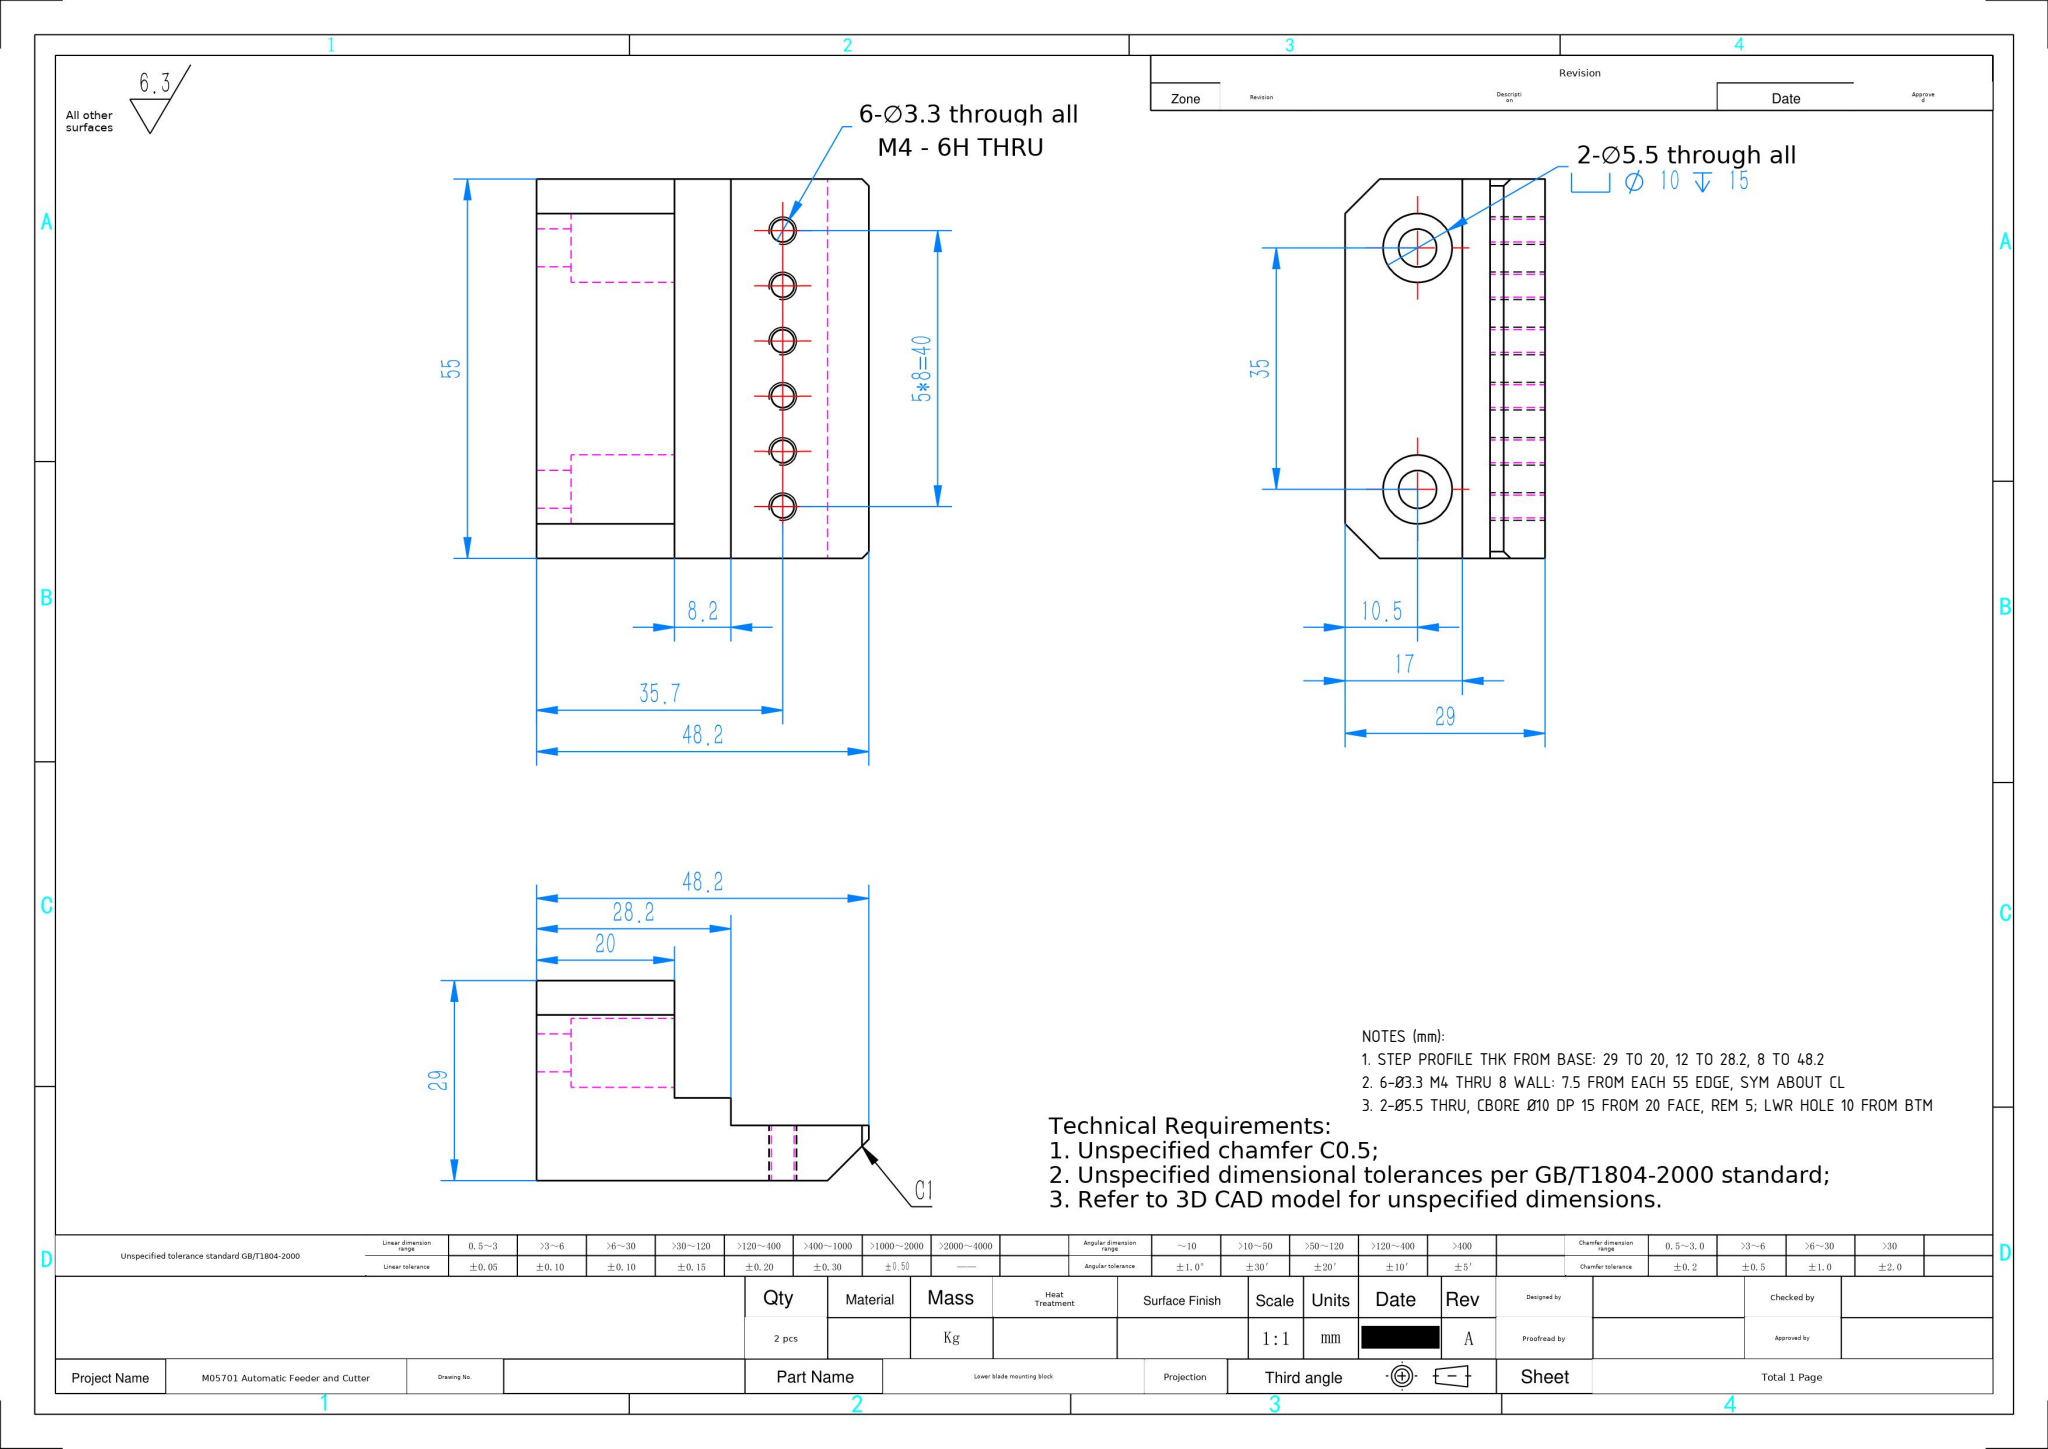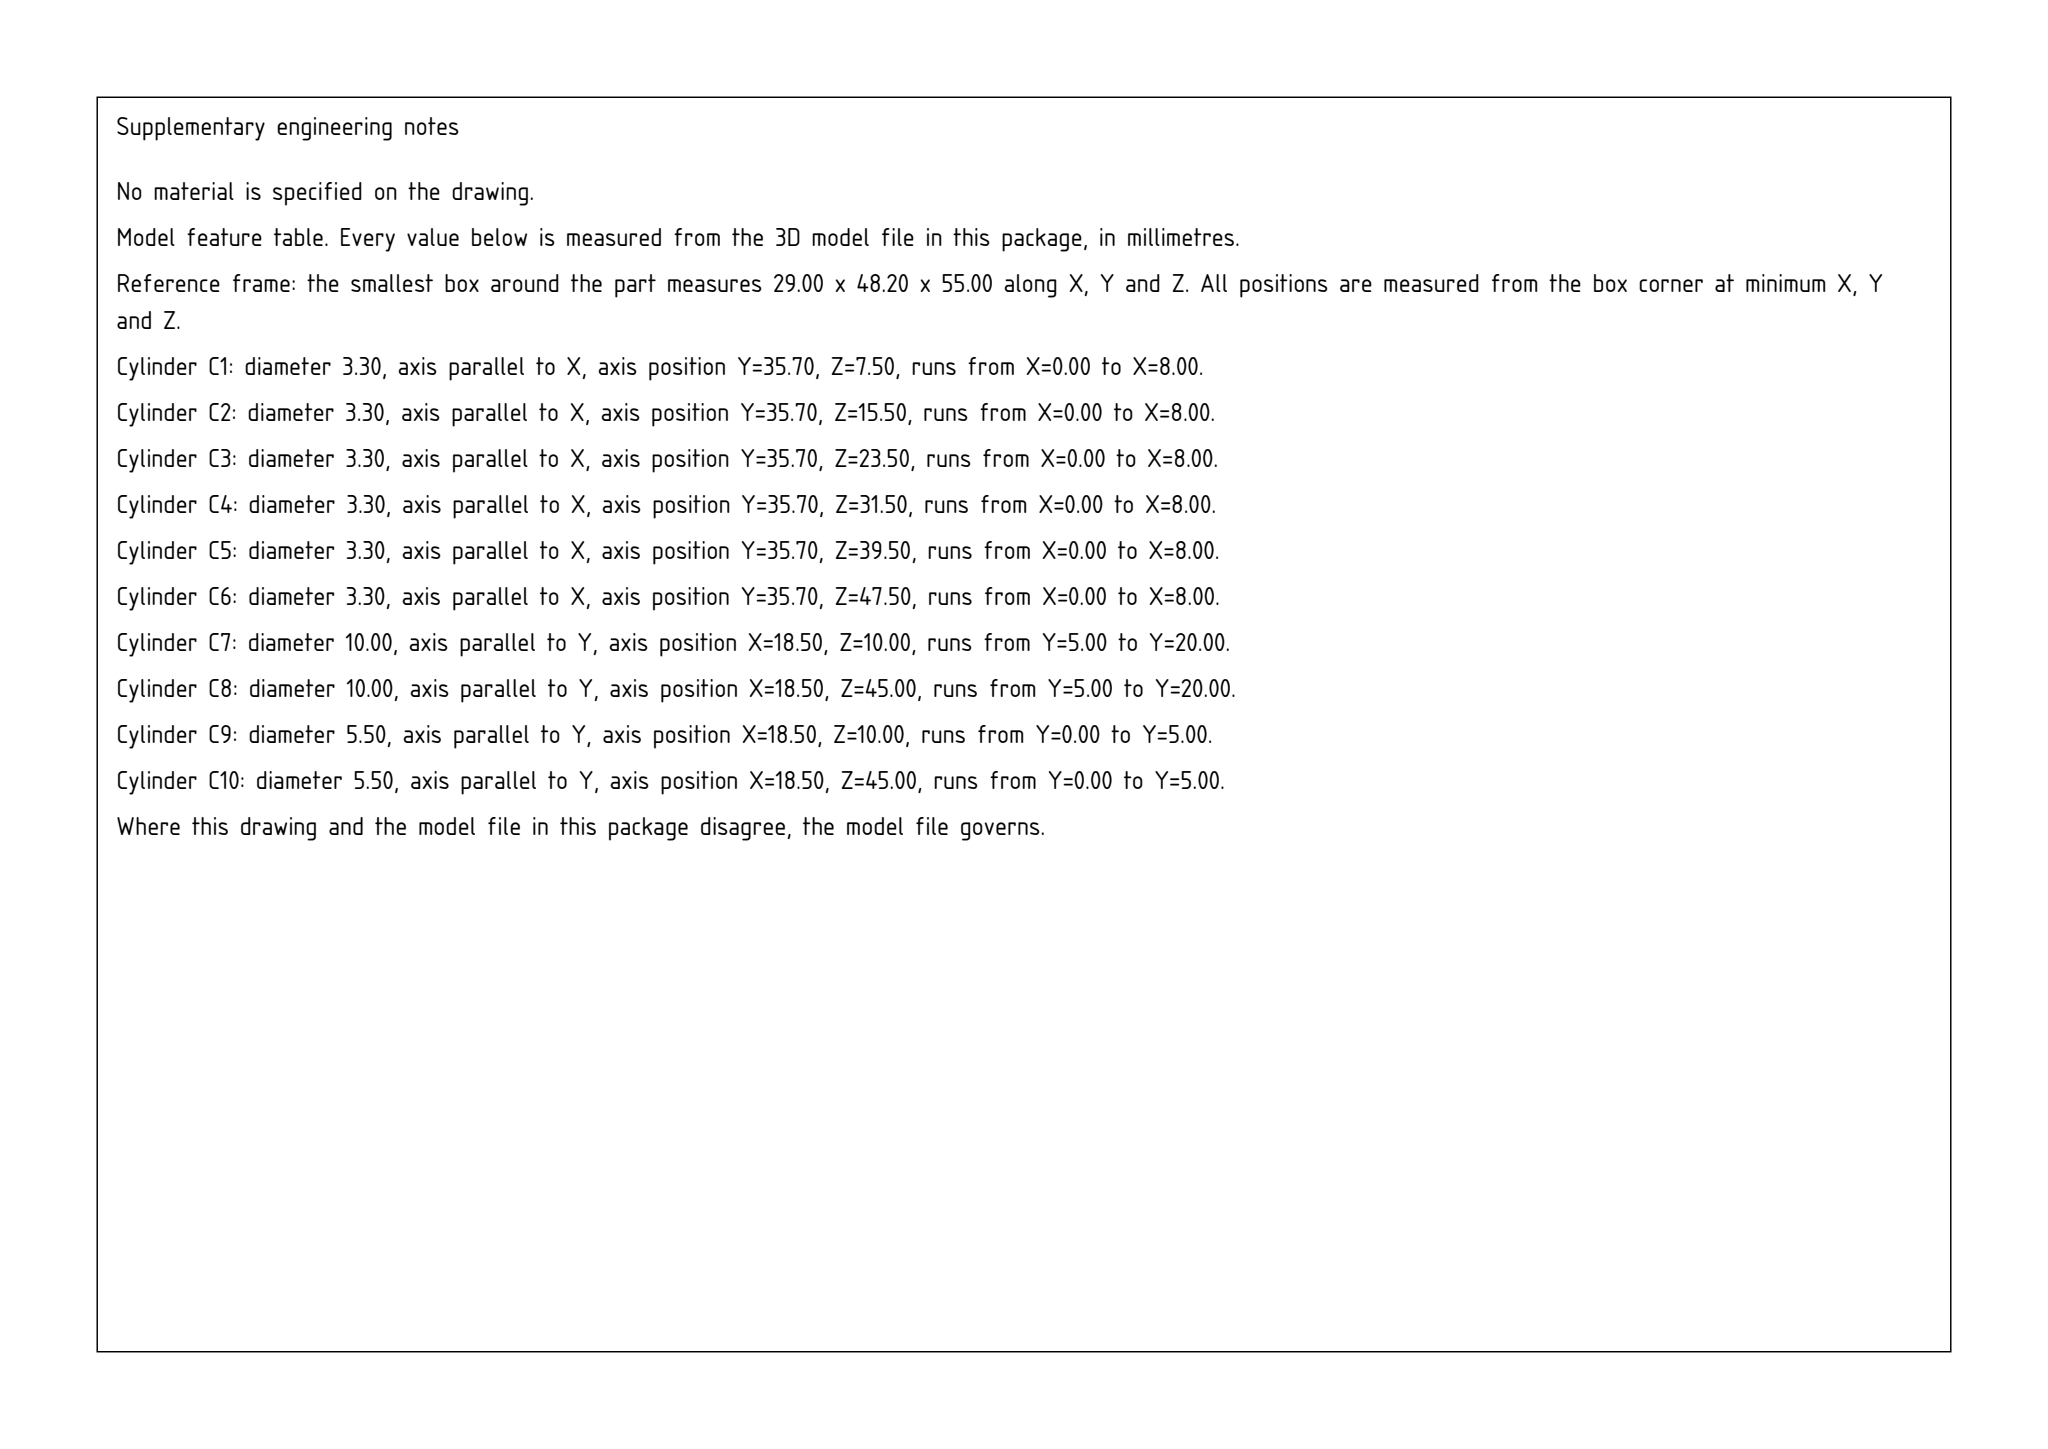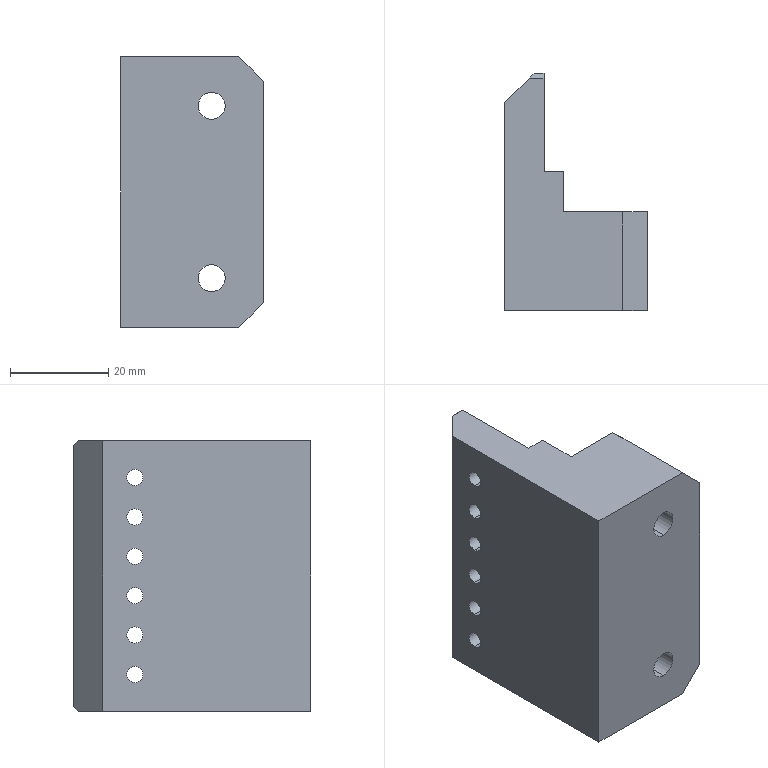Part | SolidWorks | mm | 1 solid | 37 faces | box 29 x 48.2 x 55 mm | volume 41615 mm3 | cylinder 20 | plane 17 | commonest cylinder face diameters 3.3 x12 10 x4 5.5 x4
Drawing notes:
STEP PROFILE THK FROM BASE: 29 TO 20, 12 TO 28.2, 8 TO 48.2 | from the solid: x-normal planes at 0, 8, 12, 29; y-normal planes at 20, 28.2, 48.2; bbox 29 x 48.2 x 55
6-Ø3.3 M4 THRU 8 WALL: 7.5 FROM EACH 55 EDGE, SYM ABOUT CL | from the solid: Ø3.3 axes y=35.7, z=7.5,15.5,23.5,31.5,39.5,47.5, len 8; bbox z=55, CL z=27.5
2-Ø5.5 THRU, CBORE Ø10 DP 15 FROM 20 FACE, REM 5; LWR HOLE 10 FROM BTM | from the solid: Ø10 cyl axis y len 15 + Ø5.5 axis y len 5 at x=18.5, z=10 and 45; cbore faces y=5; bbox z=55
build123d program:
from build123d import *

# Parameters (mm, degrees)
BOSS_EXTRUDE1_DEPTH                             = 55
M5_HEX_SOCKET_HEAD_CAP_SCREW_CBORE1_D           = 5.5
M5_HEX_SOCKET_HEAD_CAP_SCREW_CBORE1_CBORE_D     = 10
M5_HEX_SOCKET_HEAD_CAP_SCREW_CBORE1_CBORE_DEPTH = 15
CHAMFER1_SIZE                                   = 5
SKETCH8_W                                       = 4
SKETCH8_H                                       = 20
CUT_EXTRUDE1_DEPTH                              = 69.273
M4_TAPPED_HOLE1_D                               = 3.3
CHAMFER2_SIZE                                   = 1
CHAMFER3_SIZE                                   = 6


with BuildPart() as part:
    # Sketch1 → Boss-Extrude1 (new body)
    with BuildSketch(Plane.XY):
        Polygon((0, 0), (-17, 0), (-17, 28.2), (-29, 28.2), (-29, -20), (0, -20), align=None)
    extrude(amount=BOSS_EXTRUDE1_DEPTH)

    # M5 Hex Socket Head Cap Screw CBORE1 (through all)
    with Locations(Plane(origin=(0, 0, 0), x_dir=(1, 0, 0), z_dir=(0, 1, 0))):
        with Locations((-10.5, -10), (-10.5, -45)):
            CounterBoreHole(M5_HEX_SOCKET_HEAD_CAP_SCREW_CBORE1_D / 2, M5_HEX_SOCKET_HEAD_CAP_SCREW_CBORE1_CBORE_D / 2, M5_HEX_SOCKET_HEAD_CAP_SCREW_CBORE1_CBORE_DEPTH)

    # Chamfer1
    chamfer1_edges = [part.edges().sort_by_distance(p)[0] for p in [
        (0, -10, 55),
        (0, -10, 0),
    ]]
    chamfer(chamfer1_edges, length=CHAMFER1_SIZE)

    # Sketch8 → Cut-Extrude1 (cut, through all)
    with BuildSketch(Plane.XY.offset(55)):
        with Locations((-19, 18.2)):
            Rectangle(SKETCH8_W, SKETCH8_H)
    extrude(amount=-CUT_EXTRUDE1_DEPTH, mode=Mode.SUBTRACT)

    # M4 Tapped Hole1 (through all)
    with Locations(Plane(origin=(-21, 0, 0), x_dir=(0, 0, -1), z_dir=(1, 0, 0))):
        with Locations((-47.5, 15.7), (-7.5, 15.7), (-39.5, 15.7), (-15.5, 15.7), (-31.5, 15.7), (-23.5, 15.7)):
            Hole(M4_TAPPED_HOLE1_D / 2)

    # Chamfer2
    chamfer2_edges = [part.edges().sort_by_distance(p)[0] for p in [
        (-25, 28.2, 0),
        (-25, 28.2, 55),
    ]]
    chamfer(chamfer2_edges, length=CHAMFER2_SIZE)

    # Chamfer3
    chamfer3_edges = [part.edges().sort_by_distance(p)[0] for p in [
        (-29, 28.2, 27.5),
    ]]
    chamfer(chamfer3_edges, length=CHAMFER3_SIZE)


solid = part.part